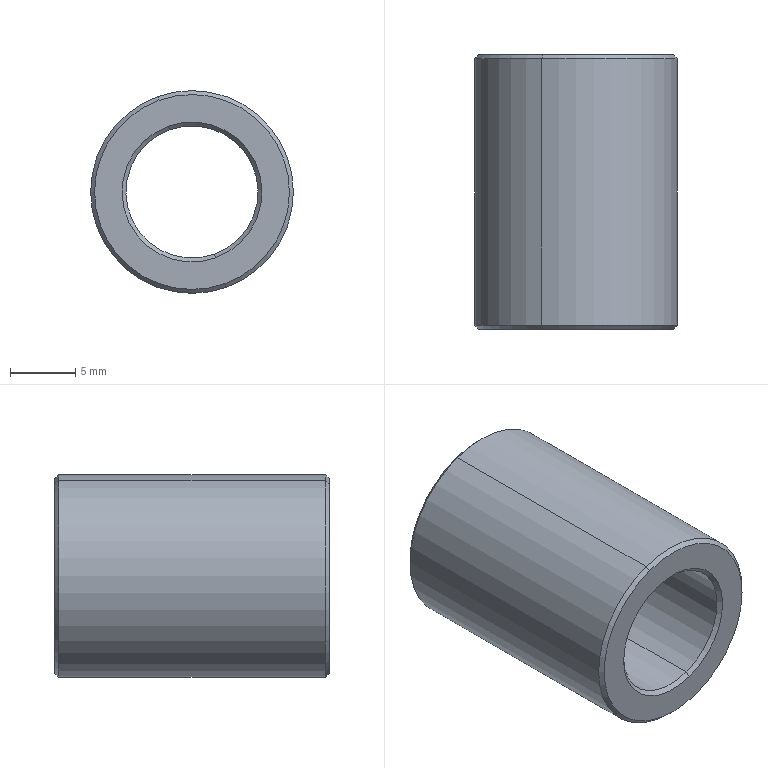Component | SolidWorks | DZ.KX.203-TC1505-30-09-01-05-30-4 | 1 solid | 14 faces | box 15.5 x 21 x 15.5 mm | volume 2273 mm3 | cone 8 | cylinder 4 | plane 2 | commonest cylinder face diameters 10.1 x2 15.5 x2
build123d program:
from build123d import *

# Parameters (mm, degrees)
SKETCH1_R           = 7.75
SKETCH1_R_2         = 5.05
BOSS_EXTRUDE1_DEPTH = 21
CHAMFER1_SIZE       = 0.3


with BuildPart() as part:
    # Sketch1 → Boss-Extrude1 (new body)
    with BuildSketch(Plane(origin=(0, 0, 0), x_dir=(0, 0, -1), z_dir=(1, 0, 0))):
        with Locations(Location((0, 0, 0), (0, 0, 180))):
            Circle(SKETCH1_R)
        with Locations(Location((0, 0, 0), (0, 0, 180))):
            Circle(SKETCH1_R_2, mode=Mode.SUBTRACT)
    extrude(amount=BOSS_EXTRUDE1_DEPTH)

    # Chamfer1
    chamfer1_edges = [part.edges().sort_by_distance(p)[0] for p in [
        (0, 0, -7.75),
        (21, 0, -7.75),
        (0, 0, -5.05),
        (21, 0, -5.05),
    ]]
    chamfer(chamfer1_edges, length=CHAMFER1_SIZE)


solid = part.part

# Placed as in the assembly
solid = solid.moved(Location((294.5, -585.807, -0.9405), (0, 0, 90)))
STEP:
#1=CARTESIAN_POINT('',(11.694,-23.063,-0.313));
#2=VERTEX_POINT('',#1);
#3=CARTESIAN_POINT('',(11.495,-23.063,0.239));
#4=VERTEX_POINT('',#3);
#5=CARTESIAN_POINT('',(11.594,-23.063,-0.03703));
#6=DIRECTION('',(0.,-1.,-0.));
#7=DIRECTION('',(-0.3386,0.,0.9409));
#8=AXIS2_PLACEMENT_3D('',#5,#6,#7);
#9=CIRCLE('',#8,0.2933);
#10=EDGE_CURVE('',#2,#4,#9,.T.);
#11=ORIENTED_EDGE('',*,*,#10,.F.);
#12=CARTESIAN_POINT('',(11.698,-23.051,-0.3241));
#13=VERTEX_POINT('',#12);
#14=CARTESIAN_POINT('',(11.698,-23.051,-0.3241));
#15=DIRECTION('',(0.2394,0.7071,-0.6653));
#16=VECTOR('',#15,39.37);
#17=LINE('',#14,#16);
#18=EDGE_CURVE('',#2,#13,#17,.T.);
#19=ORIENTED_EDGE('',*,*,#18,.T.);
#20=CARTESIAN_POINT('',(11.491,-23.051,0.2501));
#21=VERTEX_POINT('',#20);
#22=CARTESIAN_POINT('',(11.594,-23.051,-0.03703));
#23=DIRECTION('',(-0.,1.,0.));
#24=DIRECTION('',(-0.3386,0.,0.9409));
#25=AXIS2_PLACEMENT_3D('',#22,#23,#24);
#26=CIRCLE('',#25,0.3051);
#27=EDGE_CURVE('',#21,#13,#26,.T.);
#28=ORIENTED_EDGE('',*,*,#27,.F.);
#29=CARTESIAN_POINT('',(11.491,-23.051,0.2501));
#30=DIRECTION('',(-0.2394,0.7071,0.6653));
#31=VECTOR('',#30,39.37);
#32=LINE('',#29,#31);
#33=EDGE_CURVE('',#4,#21,#32,.T.);
#34=ORIENTED_EDGE('',*,*,#33,.F.);
#35=EDGE_LOOP('',(#11,#19,#28,#34));
#36=FACE_OUTER_BOUND('',#35,.T.);
#37=CARTESIAN_POINT('',(11.594,-23.051,-0.03703));
#38=DIRECTION('',(-0.,1.,0.));
#39=DIRECTION('',(-0.3386,0.,0.9409));
#40=AXIS2_PLACEMENT_3D('',#37,#38,#39);
#41=CONICAL_SURFACE('',#40,0.3051,0.7854);
#42=ADVANCED_FACE('',(#36),#41,.T.);
#43=CARTESIAN_POINT('',(11.527,-23.051,0.1501));
#44=VERTEX_POINT('',#43);
#45=CARTESIAN_POINT('',(11.662,-23.051,-0.2241));
#46=VERTEX_POINT('',#45);
#47=CARTESIAN_POINT('',(11.594,-23.051,-0.03703));
#48=DIRECTION('',(0.,-1.,-0.));
#49=DIRECTION('',(-0.3386,0.,0.9409));
#50=AXIS2_PLACEMENT_3D('',#47,#48,#49);
#51=CIRCLE('',#50,0.1988);
#52=EDGE_CURVE('',#44,#46,#51,.T.);
#53=ORIENTED_EDGE('',*,*,#52,.F.);
#54=CARTESIAN_POINT('',(11.523,-23.063,0.1612));
#55=VERTEX_POINT('',#54);
#56=CARTESIAN_POINT('',(11.523,-23.063,0.1612));
#57=DIRECTION('',(-0.2394,-0.7071,0.6653));
#58=VECTOR('',#57,39.37);
#59=LINE('',#56,#58);
#60=EDGE_CURVE('',#44,#55,#59,.T.);
#61=ORIENTED_EDGE('',*,*,#60,.T.);
#62=CARTESIAN_POINT('',(11.666,-23.063,-0.2352));
#63=VERTEX_POINT('',#62);
#64=CARTESIAN_POINT('',(11.594,-23.063,-0.03703));
#65=DIRECTION('',(-0.,1.,0.));
#66=DIRECTION('',(-0.3386,0.,0.9409));
#67=AXIS2_PLACEMENT_3D('',#64,#65,#66);
#68=CIRCLE('',#67,0.2106);
#69=EDGE_CURVE('',#63,#55,#68,.T.);
#70=ORIENTED_EDGE('',*,*,#69,.F.);
#71=CARTESIAN_POINT('',(11.666,-23.063,-0.2352));
#72=DIRECTION('',(0.2394,-0.7071,-0.6653));
#73=VECTOR('',#72,39.37);
#74=LINE('',#71,#73);
#75=EDGE_CURVE('',#46,#63,#74,.T.);
#76=ORIENTED_EDGE('',*,*,#75,.F.);
#77=EDGE_LOOP('',(#53,#61,#70,#76));
#78=FACE_OUTER_BOUND('',#77,.T.);
#79=CARTESIAN_POINT('',(11.594,-23.063,-0.03703));
#80=DIRECTION('',(0.,-1.,-0.));
#81=DIRECTION('',(0.3386,0.,-0.9409));
#82=AXIS2_PLACEMENT_3D('',#79,#80,#81);
#83=CONICAL_SURFACE('',#82,0.2106,0.7854);
#84=ADVANCED_FACE('',(#78),#83,.F.);
#85=CARTESIAN_POINT('',(11.495,-22.236,0.239));
#86=VERTEX_POINT('',#85);
#87=CARTESIAN_POINT('',(11.694,-22.236,-0.313));
#88=VERTEX_POINT('',#87);
#89=CARTESIAN_POINT('',(11.594,-22.236,-0.03703));
#90=DIRECTION('',(-0.,1.,0.));
#91=DIRECTION('',(-0.3386,0.,0.9409));
#92=AXIS2_PLACEMENT_3D('',#89,#90,#91);
#93=CIRCLE('',#92,0.2933);
#94=EDGE_CURVE('',#86,#88,#93,.T.);
#95=ORIENTED_EDGE('',*,*,#94,.F.);
#96=CARTESIAN_POINT('',(11.491,-22.248,0.2501));
#97=VERTEX_POINT('',#96);
#98=CARTESIAN_POINT('',(11.495,-22.236,0.239));
#99=DIRECTION('',(-0.2394,-0.7071,0.6653));
#100=VECTOR('',#99,39.37);
#101=LINE('',#98,#100);
#102=EDGE_CURVE('',#86,#97,#101,.T.);
#103=ORIENTED_EDGE('',*,*,#102,.T.);
#104=CARTESIAN_POINT('',(11.698,-22.248,-0.3241));
#105=VERTEX_POINT('',#104);
#106=CARTESIAN_POINT('',(11.594,-22.248,-0.03703));
#107=DIRECTION('',(0.,-1.,-0.));
#108=DIRECTION('',(-0.3386,0.,0.9409));
#109=AXIS2_PLACEMENT_3D('',#106,#107,#108);
#110=CIRCLE('',#109,0.3051);
#111=EDGE_CURVE('',#105,#97,#110,.T.);
#112=ORIENTED_EDGE('',*,*,#111,.F.);
#113=CARTESIAN_POINT('',(11.694,-22.236,-0.313));
#114=DIRECTION('',(0.2394,-0.7071,-0.6653));
#115=VECTOR('',#114,39.37);
#116=LINE('',#113,#115);
#117=EDGE_CURVE('',#88,#105,#116,.T.);
#118=ORIENTED_EDGE('',*,*,#117,.F.);
#119=EDGE_LOOP('',(#95,#103,#112,#118));
#120=FACE_OUTER_BOUND('',#119,.T.);
#121=CARTESIAN_POINT('',(11.594,-22.236,-0.03703));
#122=DIRECTION('',(0.,-1.,-0.));
#123=DIRECTION('',(0.3386,0.,-0.9409));
#124=AXIS2_PLACEMENT_3D('',#121,#122,#123);
#125=CONICAL_SURFACE('',#124,0.2933,0.7854);
#126=ADVANCED_FACE('',(#120),#125,.T.);
#127=CARTESIAN_POINT('',(11.662,-22.248,-0.2241));
#128=VERTEX_POINT('',#127);
#129=CARTESIAN_POINT('',(11.527,-22.248,0.1501));
#130=VERTEX_POINT('',#129);
#131=CARTESIAN_POINT('',(11.594,-22.248,-0.03703));
#132=DIRECTION('',(-0.,1.,0.));
#133=DIRECTION('',(-0.3386,0.,0.9409));
#134=AXIS2_PLACEMENT_3D('',#131,#132,#133);
#135=CIRCLE('',#134,0.1988);
#136=EDGE_CURVE('',#128,#130,#135,.T.);
#137=ORIENTED_EDGE('',*,*,#136,.F.);
#138=CARTESIAN_POINT('',(11.666,-22.236,-0.2352));
#139=VERTEX_POINT('',#138);
#140=CARTESIAN_POINT('',(11.662,-22.248,-0.2241));
#141=DIRECTION('',(0.2394,0.7071,-0.6653));
#142=VECTOR('',#141,39.37);
#143=LINE('',#140,#142);
#144=EDGE_CURVE('',#128,#139,#143,.T.);
#145=ORIENTED_EDGE('',*,*,#144,.T.);
#146=CARTESIAN_POINT('',(11.523,-22.236,0.1612));
#147=VERTEX_POINT('',#146);
#148=CARTESIAN_POINT('',(11.594,-22.236,-0.03703));
#149=DIRECTION('',(0.,-1.,-0.));
#150=DIRECTION('',(-0.3386,0.,0.9409));
#151=AXIS2_PLACEMENT_3D('',#148,#149,#150);
#152=CIRCLE('',#151,0.2106);
#153=EDGE_CURVE('',#147,#139,#152,.T.);
#154=ORIENTED_EDGE('',*,*,#153,.F.);
#155=CARTESIAN_POINT('',(11.527,-22.248,0.1501));
#156=DIRECTION('',(-0.2394,0.7071,0.6653));
#157=VECTOR('',#156,39.37);
#158=LINE('',#155,#157);
#159=EDGE_CURVE('',#130,#147,#158,.T.);
#160=ORIENTED_EDGE('',*,*,#159,.F.);
#161=EDGE_LOOP('',(#137,#145,#154,#160));
#162=FACE_OUTER_BOUND('',#161,.T.);
#163=CARTESIAN_POINT('',(11.594,-22.248,-0.03703));
#164=DIRECTION('',(-0.,1.,0.));
#165=DIRECTION('',(-0.3386,0.,0.9409));
#166=AXIS2_PLACEMENT_3D('',#163,#164,#165);
#167=CONICAL_SURFACE('',#166,0.1988,0.7854);
#168=ADVANCED_FACE('',(#162),#167,.F.);
#169=ORIENTED_EDGE('',*,*,#136,.T.);
#170=CARTESIAN_POINT('',(11.527,-22.236,0.1501));
#171=DIRECTION('',(0.,-1.,-0.));
#172=VECTOR('',#171,39.37);
#173=LINE('',#170,#172);
#174=EDGE_CURVE('',#130,#44,#173,.T.);
#175=ORIENTED_EDGE('',*,*,#174,.T.);
#176=ORIENTED_EDGE('',*,*,#52,.T.);
#177=CARTESIAN_POINT('',(11.662,-22.236,-0.2241));
#178=DIRECTION('',(0.,-1.,-0.));
#179=VECTOR('',#178,39.37);
#180=LINE('',#177,#179);
#181=EDGE_CURVE('',#128,#46,#180,.T.);
#182=ORIENTED_EDGE('',*,*,#181,.F.);
#183=EDGE_LOOP('',(#169,#175,#176,#182));
#184=FACE_OUTER_BOUND('',#183,.T.);
#185=CARTESIAN_POINT('',(11.594,-22.236,-0.03703));
#186=DIRECTION('',(0.,-1.,-0.));
#187=DIRECTION('',(0.3386,0.,-0.9409));
#188=AXIS2_PLACEMENT_3D('',#185,#186,#187);
#189=CYLINDRICAL_SURFACE('',#188,0.1988);
#190=ADVANCED_FACE('',(#184),#189,.F.);
#191=ORIENTED_EDGE('',*,*,#111,.T.);
#192=CARTESIAN_POINT('',(11.491,-22.236,0.2501));
#193=DIRECTION('',(0.,-1.,-0.));
#194=VECTOR('',#193,39.37);
#195=LINE('',#192,#194);
#196=EDGE_CURVE('',#97,#21,#195,.T.);
#197=ORIENTED_EDGE('',*,*,#196,.T.);
#198=ORIENTED_EDGE('',*,*,#27,.T.);
#199=CARTESIAN_POINT('',(11.698,-22.236,-0.3241));
#200=DIRECTION('',(0.,-1.,-0.));
#201=VECTOR('',#200,39.37);
#202=LINE('',#199,#201);
#203=EDGE_CURVE('',#105,#13,#202,.T.);
#204=ORIENTED_EDGE('',*,*,#203,.F.);
#205=EDGE_LOOP('',(#191,#197,#198,#204));
#206=FACE_OUTER_BOUND('',#205,.T.);
#207=CARTESIAN_POINT('',(11.594,-22.236,-0.03703));
#208=DIRECTION('',(0.,-1.,-0.));
#209=DIRECTION('',(0.3386,0.,-0.9409));
#210=AXIS2_PLACEMENT_3D('',#207,#208,#209);
#211=CYLINDRICAL_SURFACE('',#210,0.3051);
#212=ADVANCED_FACE('',(#206),#211,.T.);
#213=ORIENTED_EDGE('',*,*,#153,.T.);
#214=CARTESIAN_POINT('',(11.594,-22.236,-0.03703));
#215=DIRECTION('',(0.,-1.,-0.));
#216=DIRECTION('',(-0.3386,0.,0.9409));
#217=AXIS2_PLACEMENT_3D('',#214,#215,#216);
#218=CIRCLE('',#217,0.2106);
#219=EDGE_CURVE('',#139,#147,#218,.T.);
#220=ORIENTED_EDGE('',*,*,#219,.T.);
#221=EDGE_LOOP('',(#213,#220));
#222=FACE_BOUND('',#221,.T.);
#223=CARTESIAN_POINT('',(11.594,-22.236,-0.03703));
#224=DIRECTION('',(-0.,1.,0.));
#225=DIRECTION('',(-0.3386,0.,0.9409));
#226=AXIS2_PLACEMENT_3D('',#223,#224,#225);
#227=CIRCLE('',#226,0.2933);
#228=EDGE_CURVE('',#88,#86,#227,.T.);
#229=ORIENTED_EDGE('',*,*,#228,.T.);
#230=ORIENTED_EDGE('',*,*,#94,.T.);
#231=EDGE_LOOP('',(#229,#230));
#232=FACE_OUTER_BOUND('',#231,.T.);
#233=CARTESIAN_POINT('',(11.594,-22.236,-0.03703));
#234=DIRECTION('',(-0.,1.,0.));
#235=DIRECTION('',(-0.3386,-0.,0.9409));
#236=AXIS2_PLACEMENT_3D('',#233,#234,#235);
#237=PLANE('',#236);
#238=ADVANCED_FACE('',(#222,#232),#237,.T.);
#239=ORIENTED_EDGE('',*,*,#69,.T.);
#240=CARTESIAN_POINT('',(11.594,-23.063,-0.03703));
#241=DIRECTION('',(-0.,1.,0.));
#242=DIRECTION('',(-0.3386,0.,0.9409));
#243=AXIS2_PLACEMENT_3D('',#240,#241,#242);
#244=CIRCLE('',#243,0.2106);
#245=EDGE_CURVE('',#55,#63,#244,.T.);
#246=ORIENTED_EDGE('',*,*,#245,.T.);
#247=EDGE_LOOP('',(#239,#246));
#248=FACE_BOUND('',#247,.T.);
#249=CARTESIAN_POINT('',(11.594,-23.063,-0.03703));
#250=DIRECTION('',(0.,-1.,-0.));
#251=DIRECTION('',(-0.3386,0.,0.9409));
#252=AXIS2_PLACEMENT_3D('',#249,#250,#251);
#253=CIRCLE('',#252,0.2933);
#254=EDGE_CURVE('',#4,#2,#253,.T.);
#255=ORIENTED_EDGE('',*,*,#254,.T.);
#256=ORIENTED_EDGE('',*,*,#10,.T.);
#257=EDGE_LOOP('',(#255,#256));
#258=FACE_OUTER_BOUND('',#257,.T.);
#259=CARTESIAN_POINT('',(11.594,-23.063,-0.03703));
#260=DIRECTION('',(-0.,1.,0.));
#261=DIRECTION('',(-0.3386,-0.,0.9409));
#262=AXIS2_PLACEMENT_3D('',#259,#260,#261);
#263=PLANE('',#262);
#264=ADVANCED_FACE('',(#248,#258),#263,.F.);
#265=ORIENTED_EDGE('',*,*,#196,.F.);
#266=CARTESIAN_POINT('',(11.594,-22.248,-0.03703));
#267=DIRECTION('',(0.,-1.,-0.));
#268=DIRECTION('',(-0.3386,0.,0.9409));
#269=AXIS2_PLACEMENT_3D('',#266,#267,#268);
#270=CIRCLE('',#269,0.3051);
#271=EDGE_CURVE('',#97,#105,#270,.T.);
#272=ORIENTED_EDGE('',*,*,#271,.T.);
#273=ORIENTED_EDGE('',*,*,#203,.T.);
#274=CARTESIAN_POINT('',(11.594,-23.051,-0.03703));
#275=DIRECTION('',(-0.,1.,0.));
#276=DIRECTION('',(-0.3386,0.,0.9409));
#277=AXIS2_PLACEMENT_3D('',#274,#275,#276);
#278=CIRCLE('',#277,0.3051);
#279=EDGE_CURVE('',#13,#21,#278,.T.);
#280=ORIENTED_EDGE('',*,*,#279,.T.);
#281=EDGE_LOOP('',(#265,#272,#273,#280));
#282=FACE_OUTER_BOUND('',#281,.T.);
#283=CARTESIAN_POINT('',(11.594,-22.236,-0.03703));
#284=DIRECTION('',(0.,-1.,-0.));
#285=DIRECTION('',(0.3386,0.,-0.9409));
#286=AXIS2_PLACEMENT_3D('',#283,#284,#285);
#287=CYLINDRICAL_SURFACE('',#286,0.3051);
#288=ADVANCED_FACE('',(#282),#287,.T.);
#289=ORIENTED_EDGE('',*,*,#174,.F.);
#290=CARTESIAN_POINT('',(11.594,-22.248,-0.03703));
#291=DIRECTION('',(-0.,1.,0.));
#292=DIRECTION('',(-0.3386,0.,0.9409));
#293=AXIS2_PLACEMENT_3D('',#290,#291,#292);
#294=CIRCLE('',#293,0.1988);
#295=EDGE_CURVE('',#130,#128,#294,.T.);
#296=ORIENTED_EDGE('',*,*,#295,.T.);
#297=ORIENTED_EDGE('',*,*,#181,.T.);
#298=CARTESIAN_POINT('',(11.594,-23.051,-0.03703));
#299=DIRECTION('',(0.,-1.,-0.));
#300=DIRECTION('',(-0.3386,0.,0.9409));
#301=AXIS2_PLACEMENT_3D('',#298,#299,#300);
#302=CIRCLE('',#301,0.1988);
#303=EDGE_CURVE('',#46,#44,#302,.T.);
#304=ORIENTED_EDGE('',*,*,#303,.T.);
#305=EDGE_LOOP('',(#289,#296,#297,#304));
#306=FACE_OUTER_BOUND('',#305,.T.);
#307=CARTESIAN_POINT('',(11.594,-22.236,-0.03703));
#308=DIRECTION('',(0.,-1.,-0.));
#309=DIRECTION('',(0.3386,0.,-0.9409));
#310=AXIS2_PLACEMENT_3D('',#307,#308,#309);
#311=CYLINDRICAL_SURFACE('',#310,0.1988);
#312=ADVANCED_FACE('',(#306),#311,.F.);
#313=ORIENTED_EDGE('',*,*,#144,.F.);
#314=ORIENTED_EDGE('',*,*,#295,.F.);
#315=ORIENTED_EDGE('',*,*,#159,.T.);
#316=ORIENTED_EDGE('',*,*,#219,.F.);
#317=EDGE_LOOP('',(#313,#314,#315,#316));
#318=FACE_OUTER_BOUND('',#317,.T.);
#319=CARTESIAN_POINT('',(11.594,-22.248,-0.03703));
#320=DIRECTION('',(-0.,1.,0.));
#321=DIRECTION('',(-0.3386,0.,0.9409));
#322=AXIS2_PLACEMENT_3D('',#319,#320,#321);
#323=CONICAL_SURFACE('',#322,0.1988,0.7854);
#324=ADVANCED_FACE('',(#318),#323,.F.);
#325=ORIENTED_EDGE('',*,*,#102,.F.);
#326=ORIENTED_EDGE('',*,*,#228,.F.);
#327=ORIENTED_EDGE('',*,*,#117,.T.);
#328=ORIENTED_EDGE('',*,*,#271,.F.);
#329=EDGE_LOOP('',(#325,#326,#327,#328));
#330=FACE_OUTER_BOUND('',#329,.T.);
#331=CARTESIAN_POINT('',(11.594,-22.236,-0.03703));
#332=DIRECTION('',(0.,-1.,-0.));
#333=DIRECTION('',(0.3386,0.,-0.9409));
#334=AXIS2_PLACEMENT_3D('',#331,#332,#333);
#335=CONICAL_SURFACE('',#334,0.2933,0.7854);
#336=ADVANCED_FACE('',(#330),#335,.T.);
#337=ORIENTED_EDGE('',*,*,#60,.F.);
#338=ORIENTED_EDGE('',*,*,#303,.F.);
#339=ORIENTED_EDGE('',*,*,#75,.T.);
#340=ORIENTED_EDGE('',*,*,#245,.F.);
#341=EDGE_LOOP('',(#337,#338,#339,#340));
#342=FACE_OUTER_BOUND('',#341,.T.);
#343=CARTESIAN_POINT('',(11.594,-23.063,-0.03703));
#344=DIRECTION('',(0.,-1.,-0.));
#345=DIRECTION('',(0.3386,0.,-0.9409));
#346=AXIS2_PLACEMENT_3D('',#343,#344,#345);
#347=CONICAL_SURFACE('',#346,0.2106,0.7854);
#348=ADVANCED_FACE('',(#342),#347,.F.);
#349=ORIENTED_EDGE('',*,*,#18,.F.);
#350=ORIENTED_EDGE('',*,*,#254,.F.);
#351=ORIENTED_EDGE('',*,*,#33,.T.);
#352=ORIENTED_EDGE('',*,*,#279,.F.);
#353=EDGE_LOOP('',(#349,#350,#351,#352));
#354=FACE_OUTER_BOUND('',#353,.T.);
#355=CARTESIAN_POINT('',(11.594,-23.051,-0.03703));
#356=DIRECTION('',(-0.,1.,0.));
#357=DIRECTION('',(-0.3386,0.,0.9409));
#358=AXIS2_PLACEMENT_3D('',#355,#356,#357);
#359=CONICAL_SURFACE('',#358,0.3051,0.7854);
#360=ADVANCED_FACE('',(#354),#359,.T.);
#361=CLOSED_SHELL('',(#42,#84,#126,#168,#190,#212,#238,#264,#288,#312,#324,#336,#348,#360));
#362=MANIFOLD_SOLID_BREP('',#361);
#363=CARTESIAN_POINT('',(0.,0.,0.));
#364=DIRECTION('',(0.,0.,1.));
#365=DIRECTION('',(1.,0.,0.));
#366=AXIS2_PLACEMENT_3D('',#363,#364,#365);
#367=(LENGTH_UNIT()NAMED_UNIT(*)SI_UNIT($,.METRE.));
#368=LENGTH_MEASURE_WITH_UNIT(LENGTH_MEASURE(0.0254),#367);
#369=DIMENSIONAL_EXPONENTS(1.,0.,0.,0.,0.,0.,0.);
#370=(CONVERSION_BASED_UNIT('',#368)LENGTH_UNIT()NAMED_UNIT(#369));
#371=UNCERTAINTY_MEASURE_WITH_UNIT(LENGTH_MEASURE(0.00001),#370,'','');
#372=(NAMED_UNIT(*)PLANE_ANGLE_UNIT()SI_UNIT($,.RADIAN.));
#373=(NAMED_UNIT(*)SI_UNIT($,.STERADIAN.)SOLID_ANGLE_UNIT());
#374=(GEOMETRIC_REPRESENTATION_CONTEXT(3)GLOBAL_UNCERTAINTY_ASSIGNED_CONTEXT((#371))GLOBAL_UNIT_ASSIGNED_CONTEXT((#370,#372,#373))REPRESENTATION_CONTEXT('',''));
#375=ADVANCED_BREP_SHAPE_REPRESENTATION('',(#362,#366),#374);
#376=COLOUR_RGB('',0.7922,0.8196,0.9333);
#377=FILL_AREA_STYLE_COLOUR('',#376);
#378=FILL_AREA_STYLE('',(#377));
#379=SURFACE_STYLE_FILL_AREA(#378);
#380=SURFACE_SIDE_STYLE('',(#379));
#381=SURFACE_STYLE_USAGE(.BOTH.,#380);
#382=PRESENTATION_STYLE_ASSIGNMENT((#381));
#383=STYLED_ITEM('',(#382),#362);
#384=(LENGTH_UNIT()NAMED_UNIT(*)SI_UNIT($,.METRE.));
#385=LENGTH_MEASURE_WITH_UNIT(LENGTH_MEASURE(0.0254),#384);
#386=DIMENSIONAL_EXPONENTS(1.,0.,0.,0.,0.,0.,0.);
#387=(CONVERSION_BASED_UNIT('',#385)LENGTH_UNIT()NAMED_UNIT(#386));
#388=UNCERTAINTY_MEASURE_WITH_UNIT(LENGTH_MEASURE(0.00001),#387,'','');
#389=(NAMED_UNIT(*)PLANE_ANGLE_UNIT()SI_UNIT($,.RADIAN.));
#390=(NAMED_UNIT(*)SI_UNIT($,.STERADIAN.)SOLID_ANGLE_UNIT());
#391=(GEOMETRIC_REPRESENTATION_CONTEXT(3)GLOBAL_UNCERTAINTY_ASSIGNED_CONTEXT((#388))GLOBAL_UNIT_ASSIGNED_CONTEXT((#387,#389,#390))REPRESENTATION_CONTEXT('',''));
#392=MECHANICAL_DESIGN_GEOMETRIC_PRESENTATION_REPRESENTATION('',(#383),#391);
#393=PRESENTATION_LAYER_ASSIGNMENT('','',(#383));